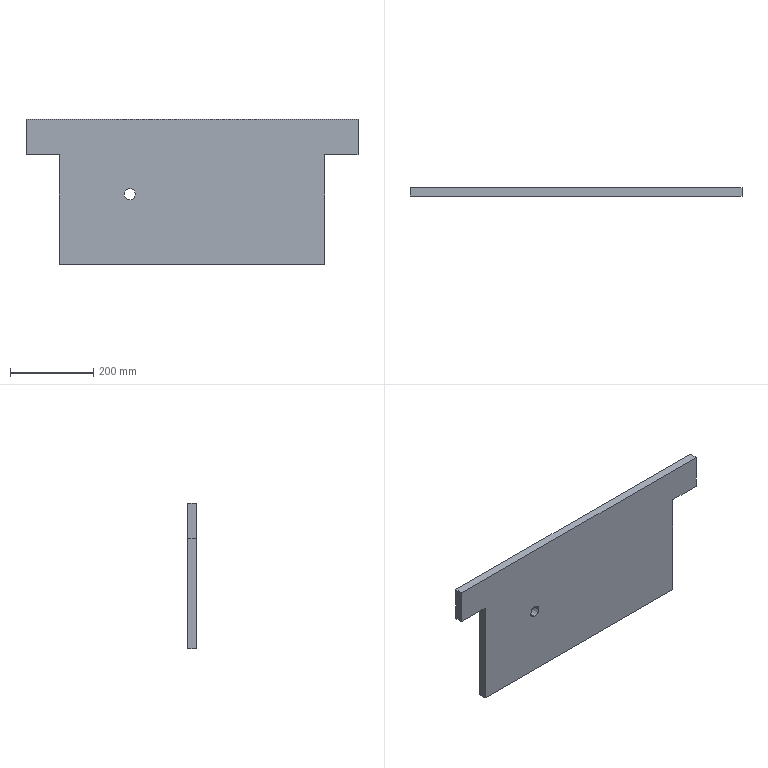Component | SolidWorks | JF21-80.1-1-3(_)-1-SOLID32-1 | 1 solid | 15 faces | box 800 x 20 x 350 mm | volume 4738255 mm3 | plane 11 | cone 2 | cylinder 2 | commonest cylinder face diameters 27 x2
STEP:
#1=COLOUR_RGB('',0.7922,0.8196,0.9333);
#2=FILL_AREA_STYLE_COLOUR('',#1);
#3=FILL_AREA_STYLE('',(#2));
#4=SURFACE_STYLE_FILL_AREA(#3);
#5=SURFACE_SIDE_STYLE('',(#4));
#6=SURFACE_STYLE_USAGE(.BOTH.,#5);
#7=PRESENTATION_STYLE_ASSIGNMENT((#6));
#8=CARTESIAN_POINT('',(-5.906,-21.067,17.341));
#9=VERTEX_POINT('',#8);
#10=CARTESIAN_POINT('',(-5.906,-21.067,18.486));
#11=VERTEX_POINT('',#10);
#12=CARTESIAN_POINT('',(-5.906,-21.067,17.913));
#13=DIRECTION('',(0.,1.,0.));
#14=DIRECTION('',(0.,0.,1.));
#15=AXIS2_PLACEMENT_3D('',#12,#13,#14);
#16=CIRCLE('',#15,0.5728);
#17=EDGE_CURVE('',#9,#11,#16,.T.);
#18=ORIENTED_EDGE('',*,*,#17,.F.);
#19=CARTESIAN_POINT('',(-5.906,-20.315,17.317));
#20=VERTEX_POINT('',#19);
#21=CARTESIAN_POINT('',(-5.906,-20.315,17.317));
#22=DIRECTION('',(0.,0.9995,-0.0312));
#23=VECTOR('',#22,39.37);
#24=LINE('',#21,#23);
#25=EDGE_CURVE('',#9,#20,#24,.T.);
#26=ORIENTED_EDGE('',*,*,#25,.T.);
#27=CARTESIAN_POINT('',(-5.906,-20.315,18.51));
#28=VERTEX_POINT('',#27);
#29=CARTESIAN_POINT('',(-5.906,-20.315,17.913));
#30=DIRECTION('',(0.,1.,0.));
#31=DIRECTION('',(0.,0.,1.));
#32=AXIS2_PLACEMENT_3D('',#29,#30,#31);
#33=CIRCLE('',#32,0.5963);
#34=EDGE_CURVE('',#20,#28,#33,.T.);
#35=ORIENTED_EDGE('',*,*,#34,.T.);
#36=CARTESIAN_POINT('',(-5.906,-20.315,18.51));
#37=DIRECTION('',(0.,0.9995,0.0312));
#38=VECTOR('',#37,39.37);
#39=LINE('',#36,#38);
#40=EDGE_CURVE('',#11,#28,#39,.T.);
#41=ORIENTED_EDGE('',*,*,#40,.F.);
#42=EDGE_LOOP('',(#18,#26,#35,#41));
#43=FACE_OUTER_BOUND('',#42,.T.);
#44=CARTESIAN_POINT('',(-5.906,-20.315,17.913));
#45=DIRECTION('',(0.,1.,0.));
#46=DIRECTION('',(0.,0.,-1.));
#47=AXIS2_PLACEMENT_3D('',#44,#45,#46);
#48=CONICAL_SURFACE('',#47,0.5963,0.03121);
#49=ADVANCED_FACE('',(#43),#48,.F.);
#50=CARTESIAN_POINT('',(-5.906,-21.102,18.445));
#51=VERTEX_POINT('',#50);
#52=CARTESIAN_POINT('',(-5.906,-21.102,17.382));
#53=VERTEX_POINT('',#52);
#54=CARTESIAN_POINT('',(-5.906,-21.102,17.913));
#55=DIRECTION('',(0.,-1.,0.));
#56=DIRECTION('',(0.,0.,-1.));
#57=AXIS2_PLACEMENT_3D('',#54,#55,#56);
#58=CIRCLE('',#57,0.5315);
#59=EDGE_CURVE('',#51,#53,#58,.T.);
#60=ORIENTED_EDGE('',*,*,#59,.T.);
#61=CARTESIAN_POINT('',(-5.906,-21.067,17.382));
#62=VERTEX_POINT('',#61);
#63=CARTESIAN_POINT('',(-5.906,-20.315,17.382));
#64=DIRECTION('',(0.,1.,0.));
#65=VECTOR('',#64,39.37);
#66=LINE('',#63,#65);
#67=EDGE_CURVE('',#53,#62,#66,.T.);
#68=ORIENTED_EDGE('',*,*,#67,.T.);
#69=CARTESIAN_POINT('',(-5.906,-21.067,18.445));
#70=VERTEX_POINT('',#69);
#71=CARTESIAN_POINT('',(-5.906,-21.067,17.913));
#72=DIRECTION('',(0.,1.,0.));
#73=DIRECTION('',(0.,0.,1.));
#74=AXIS2_PLACEMENT_3D('',#71,#72,#73);
#75=CIRCLE('',#74,0.5315);
#76=EDGE_CURVE('',#62,#70,#75,.T.);
#77=ORIENTED_EDGE('',*,*,#76,.T.);
#78=CARTESIAN_POINT('',(-5.906,-20.315,18.445));
#79=DIRECTION('',(0.,1.,0.));
#80=VECTOR('',#79,39.37);
#81=LINE('',#78,#80);
#82=EDGE_CURVE('',#51,#70,#81,.T.);
#83=ORIENTED_EDGE('',*,*,#82,.F.);
#84=EDGE_LOOP('',(#60,#68,#77,#83));
#85=FACE_OUTER_BOUND('',#84,.T.);
#86=CARTESIAN_POINT('',(-5.906,-20.315,17.913));
#87=DIRECTION('',(0.,1.,0.));
#88=DIRECTION('',(0.,0.,-1.));
#89=AXIS2_PLACEMENT_3D('',#86,#87,#88);
#90=CYLINDRICAL_SURFACE('',#89,0.5315);
#91=ADVANCED_FACE('',(#85),#90,.F.);
#92=CARTESIAN_POINT('',(-12.598,-21.102,11.22));
#93=VERTEX_POINT('',#92);
#94=CARTESIAN_POINT('',(-12.598,-21.102,21.654));
#95=VERTEX_POINT('',#94);
#96=CARTESIAN_POINT('',(-12.598,-21.102,11.22));
#97=DIRECTION('',(0.,0.,1.));
#98=VECTOR('',#97,39.37);
#99=LINE('',#96,#98);
#100=EDGE_CURVE('',#93,#95,#99,.T.);
#101=ORIENTED_EDGE('',*,*,#100,.T.);
#102=CARTESIAN_POINT('',(-12.598,-20.315,21.654));
#103=VERTEX_POINT('',#102);
#104=CARTESIAN_POINT('',(-12.598,-20.315,21.654));
#105=DIRECTION('',(0.,-1.,0.));
#106=VECTOR('',#105,39.37);
#107=LINE('',#104,#106);
#108=EDGE_CURVE('',#103,#95,#107,.T.);
#109=ORIENTED_EDGE('',*,*,#108,.F.);
#110=CARTESIAN_POINT('',(-12.598,-20.315,11.22));
#111=VERTEX_POINT('',#110);
#112=CARTESIAN_POINT('',(-12.598,-20.315,11.22));
#113=DIRECTION('',(0.,0.,1.));
#114=VECTOR('',#113,39.37);
#115=LINE('',#112,#114);
#116=EDGE_CURVE('',#111,#103,#115,.T.);
#117=ORIENTED_EDGE('',*,*,#116,.F.);
#118=CARTESIAN_POINT('',(-12.598,-20.315,11.22));
#119=DIRECTION('',(0.,-1.,0.));
#120=VECTOR('',#119,39.37);
#121=LINE('',#118,#120);
#122=EDGE_CURVE('',#111,#93,#121,.T.);
#123=ORIENTED_EDGE('',*,*,#122,.T.);
#124=EDGE_LOOP('',(#101,#109,#117,#123));
#125=FACE_OUTER_BOUND('',#124,.T.);
#126=CARTESIAN_POINT('',(-12.598,-20.315,11.22));
#127=DIRECTION('',(1.,0.,0.));
#128=DIRECTION('',(0.,0.,1.));
#129=AXIS2_PLACEMENT_3D('',#126,#127,#128);
#130=PLANE('',#129);
#131=ADVANCED_FACE('',(#125),#130,.F.);
#132=CARTESIAN_POINT('',(-15.748,-21.102,21.654));
#133=VERTEX_POINT('',#132);
#134=CARTESIAN_POINT('',(-12.598,-21.102,21.654));
#135=DIRECTION('',(-1.,0.,0.));
#136=VECTOR('',#135,39.37);
#137=LINE('',#134,#136);
#138=EDGE_CURVE('',#95,#133,#137,.T.);
#139=ORIENTED_EDGE('',*,*,#138,.T.);
#140=CARTESIAN_POINT('',(-15.748,-20.315,21.654));
#141=VERTEX_POINT('',#140);
#142=CARTESIAN_POINT('',(-15.748,-20.315,21.654));
#143=DIRECTION('',(0.,-1.,0.));
#144=VECTOR('',#143,39.37);
#145=LINE('',#142,#144);
#146=EDGE_CURVE('',#141,#133,#145,.T.);
#147=ORIENTED_EDGE('',*,*,#146,.F.);
#148=CARTESIAN_POINT('',(-12.598,-20.315,21.654));
#149=DIRECTION('',(-1.,0.,0.));
#150=VECTOR('',#149,39.37);
#151=LINE('',#148,#150);
#152=EDGE_CURVE('',#103,#141,#151,.T.);
#153=ORIENTED_EDGE('',*,*,#152,.F.);
#154=ORIENTED_EDGE('',*,*,#108,.T.);
#155=EDGE_LOOP('',(#139,#147,#153,#154));
#156=FACE_OUTER_BOUND('',#155,.T.);
#157=CARTESIAN_POINT('',(-12.598,-20.315,21.654));
#158=DIRECTION('',(0.,0.,1.));
#159=DIRECTION('',(-1.,0.,0.));
#160=AXIS2_PLACEMENT_3D('',#157,#158,#159);
#161=PLANE('',#160);
#162=ADVANCED_FACE('',(#156),#161,.F.);
#163=CARTESIAN_POINT('',(-15.748,-21.102,25.));
#164=VERTEX_POINT('',#163);
#165=CARTESIAN_POINT('',(-15.748,-21.102,25.));
#166=DIRECTION('',(0.,0.,1.));
#167=VECTOR('',#166,39.37);
#168=LINE('',#165,#167);
#169=EDGE_CURVE('',#133,#164,#168,.T.);
#170=ORIENTED_EDGE('',*,*,#169,.T.);
#171=CARTESIAN_POINT('',(-15.748,-20.315,25.));
#172=VERTEX_POINT('',#171);
#173=CARTESIAN_POINT('',(-15.748,-20.315,25.));
#174=DIRECTION('',(0.,-1.,0.));
#175=VECTOR('',#174,39.37);
#176=LINE('',#173,#175);
#177=EDGE_CURVE('',#172,#164,#176,.T.);
#178=ORIENTED_EDGE('',*,*,#177,.F.);
#179=CARTESIAN_POINT('',(-15.748,-20.315,25.));
#180=DIRECTION('',(0.,0.,1.));
#181=VECTOR('',#180,39.37);
#182=LINE('',#179,#181);
#183=EDGE_CURVE('',#141,#172,#182,.T.);
#184=ORIENTED_EDGE('',*,*,#183,.F.);
#185=ORIENTED_EDGE('',*,*,#146,.T.);
#186=EDGE_LOOP('',(#170,#178,#184,#185));
#187=FACE_OUTER_BOUND('',#186,.T.);
#188=CARTESIAN_POINT('',(-15.748,-20.315,25.));
#189=DIRECTION('',(1.,0.,0.));
#190=DIRECTION('',(0.,0.,1.));
#191=AXIS2_PLACEMENT_3D('',#188,#189,#190);
#192=PLANE('',#191);
#193=ADVANCED_FACE('',(#187),#192,.F.);
#194=CARTESIAN_POINT('',(15.748,-21.102,25.));
#195=VERTEX_POINT('',#194);
#196=CARTESIAN_POINT('',(-15.748,-21.102,25.));
#197=DIRECTION('',(1.,0.,0.));
#198=VECTOR('',#197,39.37);
#199=LINE('',#196,#198);
#200=EDGE_CURVE('',#164,#195,#199,.T.);
#201=ORIENTED_EDGE('',*,*,#200,.T.);
#202=CARTESIAN_POINT('',(15.748,-20.315,25.));
#203=VERTEX_POINT('',#202);
#204=CARTESIAN_POINT('',(15.748,-20.315,25.));
#205=DIRECTION('',(0.,-1.,0.));
#206=VECTOR('',#205,39.37);
#207=LINE('',#204,#206);
#208=EDGE_CURVE('',#203,#195,#207,.T.);
#209=ORIENTED_EDGE('',*,*,#208,.F.);
#210=CARTESIAN_POINT('',(-15.748,-20.315,25.));
#211=DIRECTION('',(1.,0.,0.));
#212=VECTOR('',#211,39.37);
#213=LINE('',#210,#212);
#214=EDGE_CURVE('',#172,#203,#213,.T.);
#215=ORIENTED_EDGE('',*,*,#214,.F.);
#216=ORIENTED_EDGE('',*,*,#177,.T.);
#217=EDGE_LOOP('',(#201,#209,#215,#216));
#218=FACE_OUTER_BOUND('',#217,.T.);
#219=CARTESIAN_POINT('',(-15.748,-20.315,25.));
#220=DIRECTION('',(0.,0.,-1.));
#221=DIRECTION('',(1.,0.,0.));
#222=AXIS2_PLACEMENT_3D('',#219,#220,#221);
#223=PLANE('',#222);
#224=ADVANCED_FACE('',(#218),#223,.F.);
#225=CARTESIAN_POINT('',(15.748,-21.102,21.654));
#226=VERTEX_POINT('',#225);
#227=CARTESIAN_POINT('',(15.748,-21.102,25.));
#228=DIRECTION('',(0.,0.,-1.));
#229=VECTOR('',#228,39.37);
#230=LINE('',#227,#229);
#231=EDGE_CURVE('',#195,#226,#230,.T.);
#232=ORIENTED_EDGE('',*,*,#231,.T.);
#233=CARTESIAN_POINT('',(15.748,-20.315,21.654));
#234=VERTEX_POINT('',#233);
#235=CARTESIAN_POINT('',(15.748,-20.315,21.654));
#236=DIRECTION('',(0.,-1.,0.));
#237=VECTOR('',#236,39.37);
#238=LINE('',#235,#237);
#239=EDGE_CURVE('',#234,#226,#238,.T.);
#240=ORIENTED_EDGE('',*,*,#239,.F.);
#241=CARTESIAN_POINT('',(15.748,-20.315,25.));
#242=DIRECTION('',(0.,0.,-1.));
#243=VECTOR('',#242,39.37);
#244=LINE('',#241,#243);
#245=EDGE_CURVE('',#203,#234,#244,.T.);
#246=ORIENTED_EDGE('',*,*,#245,.F.);
#247=ORIENTED_EDGE('',*,*,#208,.T.);
#248=EDGE_LOOP('',(#232,#240,#246,#247));
#249=FACE_OUTER_BOUND('',#248,.T.);
#250=CARTESIAN_POINT('',(15.748,-20.315,25.));
#251=DIRECTION('',(-1.,0.,0.));
#252=DIRECTION('',(0.,0.,-1.));
#253=AXIS2_PLACEMENT_3D('',#250,#251,#252);
#254=PLANE('',#253);
#255=ADVANCED_FACE('',(#249),#254,.F.);
#256=CARTESIAN_POINT('',(12.598,-21.102,21.654));
#257=VERTEX_POINT('',#256);
#258=CARTESIAN_POINT('',(12.598,-21.102,21.654));
#259=DIRECTION('',(-1.,0.,0.));
#260=VECTOR('',#259,39.37);
#261=LINE('',#258,#260);
#262=EDGE_CURVE('',#226,#257,#261,.T.);
#263=ORIENTED_EDGE('',*,*,#262,.T.);
#264=CARTESIAN_POINT('',(12.598,-20.315,21.654));
#265=VERTEX_POINT('',#264);
#266=CARTESIAN_POINT('',(12.598,-20.315,21.654));
#267=DIRECTION('',(0.,-1.,0.));
#268=VECTOR('',#267,39.37);
#269=LINE('',#266,#268);
#270=EDGE_CURVE('',#265,#257,#269,.T.);
#271=ORIENTED_EDGE('',*,*,#270,.F.);
#272=CARTESIAN_POINT('',(12.598,-20.315,21.654));
#273=DIRECTION('',(-1.,0.,0.));
#274=VECTOR('',#273,39.37);
#275=LINE('',#272,#274);
#276=EDGE_CURVE('',#234,#265,#275,.T.);
#277=ORIENTED_EDGE('',*,*,#276,.F.);
#278=ORIENTED_EDGE('',*,*,#239,.T.);
#279=EDGE_LOOP('',(#263,#271,#277,#278));
#280=FACE_OUTER_BOUND('',#279,.T.);
#281=CARTESIAN_POINT('',(12.598,-20.315,21.654));
#282=DIRECTION('',(0.,0.,1.));
#283=DIRECTION('',(-1.,0.,0.));
#284=AXIS2_PLACEMENT_3D('',#281,#282,#283);
#285=PLANE('',#284);
#286=ADVANCED_FACE('',(#280),#285,.F.);
#287=CARTESIAN_POINT('',(12.598,-21.102,11.22));
#288=VERTEX_POINT('',#287);
#289=CARTESIAN_POINT('',(12.598,-21.102,11.22));
#290=DIRECTION('',(0.,0.,-1.));
#291=VECTOR('',#290,39.37);
#292=LINE('',#289,#291);
#293=EDGE_CURVE('',#257,#288,#292,.T.);
#294=ORIENTED_EDGE('',*,*,#293,.T.);
#295=CARTESIAN_POINT('',(12.598,-20.315,11.22));
#296=VERTEX_POINT('',#295);
#297=CARTESIAN_POINT('',(12.598,-20.315,11.22));
#298=DIRECTION('',(0.,-1.,0.));
#299=VECTOR('',#298,39.37);
#300=LINE('',#297,#299);
#301=EDGE_CURVE('',#296,#288,#300,.T.);
#302=ORIENTED_EDGE('',*,*,#301,.F.);
#303=CARTESIAN_POINT('',(12.598,-20.315,11.22));
#304=DIRECTION('',(0.,0.,-1.));
#305=VECTOR('',#304,39.37);
#306=LINE('',#303,#305);
#307=EDGE_CURVE('',#265,#296,#306,.T.);
#308=ORIENTED_EDGE('',*,*,#307,.F.);
#309=ORIENTED_EDGE('',*,*,#270,.T.);
#310=EDGE_LOOP('',(#294,#302,#308,#309));
#311=FACE_OUTER_BOUND('',#310,.T.);
#312=CARTESIAN_POINT('',(12.598,-20.315,11.22));
#313=DIRECTION('',(-1.,0.,0.));
#314=DIRECTION('',(0.,0.,-1.));
#315=AXIS2_PLACEMENT_3D('',#312,#313,#314);
#316=PLANE('',#315);
#317=ADVANCED_FACE('',(#311),#316,.F.);
#318=CARTESIAN_POINT('',(-12.598,-21.102,11.22));
#319=DIRECTION('',(-1.,0.,0.));
#320=VECTOR('',#319,39.37);
#321=LINE('',#318,#320);
#322=EDGE_CURVE('',#288,#93,#321,.T.);
#323=ORIENTED_EDGE('',*,*,#322,.T.);
#324=ORIENTED_EDGE('',*,*,#122,.F.);
#325=CARTESIAN_POINT('',(-12.598,-20.315,11.22));
#326=DIRECTION('',(-1.,0.,0.));
#327=VECTOR('',#326,39.37);
#328=LINE('',#325,#327);
#329=EDGE_CURVE('',#296,#111,#328,.T.);
#330=ORIENTED_EDGE('',*,*,#329,.F.);
#331=ORIENTED_EDGE('',*,*,#301,.T.);
#332=EDGE_LOOP('',(#323,#324,#330,#331));
#333=FACE_OUTER_BOUND('',#332,.T.);
#334=CARTESIAN_POINT('',(-12.598,-20.315,11.22));
#335=DIRECTION('',(0.,0.,1.));
#336=DIRECTION('',(-1.,0.,0.));
#337=AXIS2_PLACEMENT_3D('',#334,#335,#336);
#338=PLANE('',#337);
#339=ADVANCED_FACE('',(#333),#338,.F.);
#340=CARTESIAN_POINT('',(-5.906,-20.315,17.913));
#341=DIRECTION('',(0.,1.,0.));
#342=DIRECTION('',(0.,0.,1.));
#343=AXIS2_PLACEMENT_3D('',#340,#341,#342);
#344=CIRCLE('',#343,0.5963);
#345=EDGE_CURVE('',#28,#20,#344,.T.);
#346=ORIENTED_EDGE('',*,*,#345,.F.);
#347=ORIENTED_EDGE('',*,*,#34,.F.);
#348=EDGE_LOOP('',(#346,#347));
#349=FACE_BOUND('',#348,.T.);
#350=ORIENTED_EDGE('',*,*,#116,.T.);
#351=ORIENTED_EDGE('',*,*,#152,.T.);
#352=ORIENTED_EDGE('',*,*,#183,.T.);
#353=ORIENTED_EDGE('',*,*,#214,.T.);
#354=ORIENTED_EDGE('',*,*,#245,.T.);
#355=ORIENTED_EDGE('',*,*,#276,.T.);
#356=ORIENTED_EDGE('',*,*,#307,.T.);
#357=ORIENTED_EDGE('',*,*,#329,.T.);
#358=EDGE_LOOP('',(#350,#351,#352,#353,#354,#355,#356,#357));
#359=FACE_OUTER_BOUND('',#358,.T.);
#360=CARTESIAN_POINT('',(-12.598,-20.315,21.654));
#361=DIRECTION('',(0.,-1.,0.));
#362=DIRECTION('',(0.,0.,1.));
#363=AXIS2_PLACEMENT_3D('',#360,#361,#362);
#364=PLANE('',#363);
#365=ADVANCED_FACE('',(#349,#359),#364,.F.);
#366=ORIENTED_EDGE('',*,*,#59,.F.);
#367=CARTESIAN_POINT('',(-5.906,-21.102,17.913));
#368=DIRECTION('',(0.,-1.,0.));
#369=DIRECTION('',(0.,0.,-1.));
#370=AXIS2_PLACEMENT_3D('',#367,#368,#369);
#371=CIRCLE('',#370,0.5315);
#372=EDGE_CURVE('',#53,#51,#371,.T.);
#373=ORIENTED_EDGE('',*,*,#372,.F.);
#374=EDGE_LOOP('',(#366,#373));
#375=FACE_BOUND('',#374,.T.);
#376=ORIENTED_EDGE('',*,*,#100,.F.);
#377=ORIENTED_EDGE('',*,*,#322,.F.);
#378=ORIENTED_EDGE('',*,*,#293,.F.);
#379=ORIENTED_EDGE('',*,*,#262,.F.);
#380=ORIENTED_EDGE('',*,*,#231,.F.);
#381=ORIENTED_EDGE('',*,*,#200,.F.);
#382=ORIENTED_EDGE('',*,*,#169,.F.);
#383=ORIENTED_EDGE('',*,*,#138,.F.);
#384=EDGE_LOOP('',(#376,#377,#378,#379,#380,#381,#382,#383));
#385=FACE_OUTER_BOUND('',#384,.T.);
#386=CARTESIAN_POINT('',(-12.598,-21.102,21.654));
#387=DIRECTION('',(0.,-1.,0.));
#388=DIRECTION('',(0.,0.,1.));
#389=AXIS2_PLACEMENT_3D('',#386,#387,#388);
#390=PLANE('',#389);
#391=ADVANCED_FACE('',(#375,#385),#390,.T.);
#392=ORIENTED_EDGE('',*,*,#67,.F.);
#393=ORIENTED_EDGE('',*,*,#372,.T.);
#394=ORIENTED_EDGE('',*,*,#82,.T.);
#395=CARTESIAN_POINT('',(-5.906,-21.067,17.913));
#396=DIRECTION('',(0.,1.,0.));
#397=DIRECTION('',(0.,0.,1.));
#398=AXIS2_PLACEMENT_3D('',#395,#396,#397);
#399=CIRCLE('',#398,0.5315);
#400=EDGE_CURVE('',#70,#62,#399,.T.);
#401=ORIENTED_EDGE('',*,*,#400,.T.);
#402=EDGE_LOOP('',(#392,#393,#394,#401));
#403=FACE_OUTER_BOUND('',#402,.T.);
#404=CARTESIAN_POINT('',(-5.906,-20.315,17.913));
#405=DIRECTION('',(0.,1.,0.));
#406=DIRECTION('',(0.,0.,-1.));
#407=AXIS2_PLACEMENT_3D('',#404,#405,#406);
#408=CYLINDRICAL_SURFACE('',#407,0.5315);
#409=ADVANCED_FACE('',(#403),#408,.F.);
#410=ORIENTED_EDGE('',*,*,#400,.F.);
#411=ORIENTED_EDGE('',*,*,#76,.F.);
#412=EDGE_LOOP('',(#410,#411));
#413=FACE_BOUND('',#412,.T.);
#414=CARTESIAN_POINT('',(-5.906,-21.067,17.913));
#415=DIRECTION('',(0.,1.,0.));
#416=DIRECTION('',(0.,0.,1.));
#417=AXIS2_PLACEMENT_3D('',#414,#415,#416);
#418=CIRCLE('',#417,0.5728);
#419=EDGE_CURVE('',#11,#9,#418,.T.);
#420=ORIENTED_EDGE('',*,*,#419,.T.);
#421=ORIENTED_EDGE('',*,*,#17,.T.);
#422=EDGE_LOOP('',(#420,#421));
#423=FACE_OUTER_BOUND('',#422,.T.);
#424=CARTESIAN_POINT('',(-5.374,-21.067,17.913));
#425=DIRECTION('',(0.,-1.,0.));
#426=DIRECTION('',(0.,0.,1.));
#427=AXIS2_PLACEMENT_3D('',#424,#425,#426);
#428=PLANE('',#427);
#429=ADVANCED_FACE('',(#413,#423),#428,.F.);
#430=ORIENTED_EDGE('',*,*,#25,.F.);
#431=ORIENTED_EDGE('',*,*,#419,.F.);
#432=ORIENTED_EDGE('',*,*,#40,.T.);
#433=ORIENTED_EDGE('',*,*,#345,.T.);
#434=EDGE_LOOP('',(#430,#431,#432,#433));
#435=FACE_OUTER_BOUND('',#434,.T.);
#436=CARTESIAN_POINT('',(-5.906,-20.315,17.913));
#437=DIRECTION('',(0.,1.,0.));
#438=DIRECTION('',(0.,0.,-1.));
#439=AXIS2_PLACEMENT_3D('',#436,#437,#438);
#440=CONICAL_SURFACE('',#439,0.5963,0.03121);
#441=ADVANCED_FACE('',(#435),#440,.F.);
#442=CLOSED_SHELL('',(#49,#91,#131,#162,#193,#224,#255,#286,#317,#339,#365,#391,#409,#429,#441));
#443=MANIFOLD_SOLID_BREP('',#442);
#444=STYLED_ITEM('',(#7),#443);
#445=PRESENTATION_LAYER_ASSIGNMENT('','',(#444));
#446=(LENGTH_UNIT()NAMED_UNIT(*)SI_UNIT($,.METRE.));
#447=LENGTH_MEASURE_WITH_UNIT(LENGTH_MEASURE(0.0254),#446);
#448=DIMENSIONAL_EXPONENTS(1.,0.,0.,0.,0.,0.,0.);
#449=(CONVERSION_BASED_UNIT('',#447)LENGTH_UNIT()NAMED_UNIT(#448));
#450=UNCERTAINTY_MEASURE_WITH_UNIT(LENGTH_MEASURE(0.00001),#449,'','');
#451=(NAMED_UNIT(*)PLANE_ANGLE_UNIT()SI_UNIT($,.RADIAN.));
#452=(NAMED_UNIT(*)SI_UNIT($,.STERADIAN.)SOLID_ANGLE_UNIT());
#453=(GEOMETRIC_REPRESENTATION_CONTEXT(3)GLOBAL_UNCERTAINTY_ASSIGNED_CONTEXT((#450))GLOBAL_UNIT_ASSIGNED_CONTEXT((#449,#451,#452))REPRESENTATION_CONTEXT('',''));
#454=MECHANICAL_DESIGN_GEOMETRIC_PRESENTATION_REPRESENTATION('',(#444),#453);
#455=CARTESIAN_POINT('',(0.,0.,0.));
#456=DIRECTION('',(0.,0.,1.));
#457=DIRECTION('',(1.,0.,0.));
#458=AXIS2_PLACEMENT_3D('',#455,#456,#457);
#459=(LENGTH_UNIT()NAMED_UNIT(*)SI_UNIT($,.METRE.));
#460=LENGTH_MEASURE_WITH_UNIT(LENGTH_MEASURE(0.0254),#459);
#461=DIMENSIONAL_EXPONENTS(1.,0.,0.,0.,0.,0.,0.);
#462=(CONVERSION_BASED_UNIT('',#460)LENGTH_UNIT()NAMED_UNIT(#461));
#463=UNCERTAINTY_MEASURE_WITH_UNIT(LENGTH_MEASURE(0.00001),#462,'','');
#464=(NAMED_UNIT(*)PLANE_ANGLE_UNIT()SI_UNIT($,.RADIAN.));
#465=(NAMED_UNIT(*)SI_UNIT($,.STERADIAN.)SOLID_ANGLE_UNIT());
#466=(GEOMETRIC_REPRESENTATION_CONTEXT(3)GLOBAL_UNCERTAINTY_ASSIGNED_CONTEXT((#463))GLOBAL_UNIT_ASSIGNED_CONTEXT((#462,#464,#465))REPRESENTATION_CONTEXT('',''));
#467=ADVANCED_BREP_SHAPE_REPRESENTATION('',(#443,#458),#466);